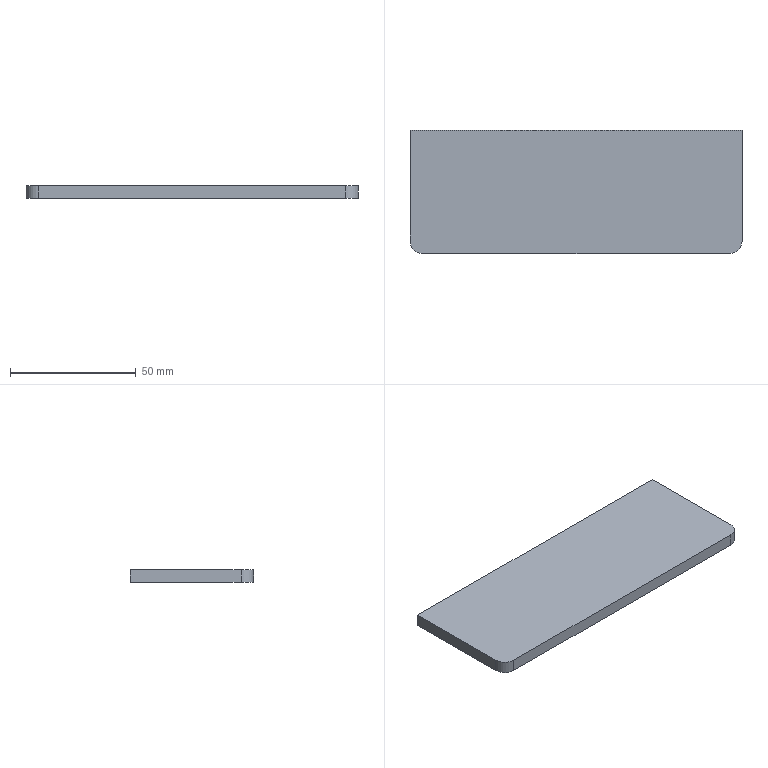Component | SolidWorks | LiftingVerticalBeamAssembly-1_LiftingVerticalBeamStiffener-2 | 1 solid | 8 faces | box 132 x 49 x 5 mm | volume 32286 mm3 | plane 6 | cylinder 2 | commonest cylinder face diameters 10 x2 | material Plain Carbon Steel
STEP:
#1=COLOUR_RGB('',0.7922,0.8196,0.9333);
#2=FILL_AREA_STYLE_COLOUR('',#1);
#3=FILL_AREA_STYLE('',(#2));
#4=SURFACE_STYLE_FILL_AREA(#3);
#5=SURFACE_SIDE_STYLE('',(#4));
#6=SURFACE_STYLE_USAGE(.BOTH.,#5);
#7=PRESENTATION_STYLE_ASSIGNMENT((#6));
#8=CARTESIAN_POINT('',(69.027,0.7303,53.05));
#9=VERTEX_POINT('',#8);
#10=CARTESIAN_POINT('',(69.027,-1.002,53.05));
#11=VERTEX_POINT('',#10);
#12=CARTESIAN_POINT('',(69.027,0.7303,53.05));
#13=DIRECTION('',(0.,-1.,0.));
#14=VECTOR('',#13,39.37);
#15=LINE('',#12,#14);
#16=EDGE_CURVE('',#9,#11,#15,.T.);
#17=ORIENTED_EDGE('',*,*,#16,.T.);
#18=CARTESIAN_POINT('',(69.027,-1.002,53.247));
#19=VERTEX_POINT('',#18);
#20=CARTESIAN_POINT('',(69.027,-1.002,53.05));
#21=DIRECTION('',(0.,0.,1.));
#22=VECTOR('',#21,39.37);
#23=LINE('',#20,#22);
#24=EDGE_CURVE('',#11,#19,#23,.T.);
#25=ORIENTED_EDGE('',*,*,#24,.T.);
#26=CARTESIAN_POINT('',(69.027,0.7303,53.247));
#27=VERTEX_POINT('',#26);
#28=CARTESIAN_POINT('',(69.027,0.7303,53.247));
#29=DIRECTION('',(0.,-1.,0.));
#30=VECTOR('',#29,39.37);
#31=LINE('',#28,#30);
#32=EDGE_CURVE('',#27,#19,#31,.T.);
#33=ORIENTED_EDGE('',*,*,#32,.F.);
#34=CARTESIAN_POINT('',(69.027,0.7303,53.05));
#35=DIRECTION('',(0.,0.,1.));
#36=VECTOR('',#35,39.37);
#37=LINE('',#34,#36);
#38=EDGE_CURVE('',#9,#27,#37,.T.);
#39=ORIENTED_EDGE('',*,*,#38,.F.);
#40=EDGE_LOOP('',(#17,#25,#33,#39));
#41=FACE_OUTER_BOUND('',#40,.T.);
#42=CARTESIAN_POINT('',(69.027,0.7303,53.05));
#43=DIRECTION('',(-1.,-0.,0.));
#44=DIRECTION('',(0.,-1.,0.));
#45=AXIS2_PLACEMENT_3D('',#42,#43,#44);
#46=PLANE('',#45);
#47=ADVANCED_FACE('',(#41),#46,.T.);
#48=CARTESIAN_POINT('',(74.224,0.7303,53.247));
#49=VERTEX_POINT('',#48);
#50=CARTESIAN_POINT('',(69.027,0.7303,53.247));
#51=DIRECTION('',(-1.,0.,0.));
#52=VECTOR('',#51,39.37);
#53=LINE('',#50,#52);
#54=EDGE_CURVE('',#49,#27,#53,.T.);
#55=ORIENTED_EDGE('',*,*,#54,.F.);
#56=CARTESIAN_POINT('',(74.224,0.7303,53.05));
#57=VERTEX_POINT('',#56);
#58=CARTESIAN_POINT('',(74.224,0.7303,53.05));
#59=DIRECTION('',(0.,0.,1.));
#60=VECTOR('',#59,39.37);
#61=LINE('',#58,#60);
#62=EDGE_CURVE('',#57,#49,#61,.T.);
#63=ORIENTED_EDGE('',*,*,#62,.F.);
#64=CARTESIAN_POINT('',(69.027,0.7303,53.05));
#65=DIRECTION('',(-1.,0.,0.));
#66=VECTOR('',#65,39.37);
#67=LINE('',#64,#66);
#68=EDGE_CURVE('',#57,#9,#67,.T.);
#69=ORIENTED_EDGE('',*,*,#68,.T.);
#70=ORIENTED_EDGE('',*,*,#38,.T.);
#71=EDGE_LOOP('',(#55,#63,#69,#70));
#72=FACE_OUTER_BOUND('',#71,.T.);
#73=CARTESIAN_POINT('',(69.027,0.7303,53.05));
#74=DIRECTION('',(0.,1.,0.));
#75=DIRECTION('',(0.,0.,1.));
#76=AXIS2_PLACEMENT_3D('',#73,#74,#75);
#77=PLANE('',#76);
#78=ADVANCED_FACE('',(#72),#77,.T.);
#79=CARTESIAN_POINT('',(74.224,-1.002,53.247));
#80=VERTEX_POINT('',#79);
#81=CARTESIAN_POINT('',(74.224,0.7303,53.247));
#82=DIRECTION('',(0.,1.,0.));
#83=VECTOR('',#82,39.37);
#84=LINE('',#81,#83);
#85=EDGE_CURVE('',#80,#49,#84,.T.);
#86=ORIENTED_EDGE('',*,*,#85,.F.);
#87=CARTESIAN_POINT('',(74.224,-1.002,53.05));
#88=VERTEX_POINT('',#87);
#89=CARTESIAN_POINT('',(74.224,-1.002,53.05));
#90=DIRECTION('',(0.,0.,-1.));
#91=VECTOR('',#90,39.37);
#92=LINE('',#89,#91);
#93=EDGE_CURVE('',#80,#88,#92,.T.);
#94=ORIENTED_EDGE('',*,*,#93,.T.);
#95=CARTESIAN_POINT('',(74.224,0.7303,53.05));
#96=DIRECTION('',(0.,1.,0.));
#97=VECTOR('',#96,39.37);
#98=LINE('',#95,#97);
#99=EDGE_CURVE('',#88,#57,#98,.T.);
#100=ORIENTED_EDGE('',*,*,#99,.T.);
#101=ORIENTED_EDGE('',*,*,#62,.T.);
#102=EDGE_LOOP('',(#86,#94,#100,#101));
#103=FACE_OUTER_BOUND('',#102,.T.);
#104=CARTESIAN_POINT('',(74.224,0.7303,53.05));
#105=DIRECTION('',(1.,0.,0.));
#106=DIRECTION('',(0.,0.,-1.));
#107=AXIS2_PLACEMENT_3D('',#104,#105,#106);
#108=PLANE('',#107);
#109=ADVANCED_FACE('',(#103),#108,.T.);
#110=CARTESIAN_POINT('',(69.224,-1.199,53.05));
#111=VERTEX_POINT('',#110);
#112=CARTESIAN_POINT('',(74.027,-1.199,53.05));
#113=VERTEX_POINT('',#112);
#114=CARTESIAN_POINT('',(69.027,-1.199,53.05));
#115=DIRECTION('',(1.,0.,0.));
#116=VECTOR('',#115,39.37);
#117=LINE('',#114,#116);
#118=EDGE_CURVE('',#111,#113,#117,.T.);
#119=ORIENTED_EDGE('',*,*,#118,.T.);
#120=CARTESIAN_POINT('',(74.027,-1.199,53.247));
#121=VERTEX_POINT('',#120);
#122=CARTESIAN_POINT('',(74.027,-1.199,53.05));
#123=DIRECTION('',(0.,0.,1.));
#124=VECTOR('',#123,39.37);
#125=LINE('',#122,#124);
#126=EDGE_CURVE('',#113,#121,#125,.T.);
#127=ORIENTED_EDGE('',*,*,#126,.T.);
#128=CARTESIAN_POINT('',(69.224,-1.199,53.247));
#129=VERTEX_POINT('',#128);
#130=CARTESIAN_POINT('',(69.027,-1.199,53.247));
#131=DIRECTION('',(1.,0.,0.));
#132=VECTOR('',#131,39.37);
#133=LINE('',#130,#132);
#134=EDGE_CURVE('',#129,#121,#133,.T.);
#135=ORIENTED_EDGE('',*,*,#134,.F.);
#136=CARTESIAN_POINT('',(69.224,-1.199,53.05));
#137=DIRECTION('',(0.,0.,-1.));
#138=VECTOR('',#137,39.37);
#139=LINE('',#136,#138);
#140=EDGE_CURVE('',#129,#111,#139,.T.);
#141=ORIENTED_EDGE('',*,*,#140,.T.);
#142=EDGE_LOOP('',(#119,#127,#135,#141));
#143=FACE_OUTER_BOUND('',#142,.T.);
#144=CARTESIAN_POINT('',(69.027,-1.199,53.05));
#145=DIRECTION('',(0.,-1.,0.));
#146=DIRECTION('',(0.,0.,-1.));
#147=AXIS2_PLACEMENT_3D('',#144,#145,#146);
#148=PLANE('',#147);
#149=ADVANCED_FACE('',(#143),#148,.T.);
#150=ORIENTED_EDGE('',*,*,#99,.F.);
#151=CARTESIAN_POINT('',(74.027,-1.002,53.05));
#152=DIRECTION('',(0.,0.,-1.));
#153=DIRECTION('',(1.,0.,0.));
#154=AXIS2_PLACEMENT_3D('',#151,#152,#153);
#155=CIRCLE('',#154,0.1969);
#156=EDGE_CURVE('',#88,#113,#155,.T.);
#157=ORIENTED_EDGE('',*,*,#156,.T.);
#158=ORIENTED_EDGE('',*,*,#118,.F.);
#159=CARTESIAN_POINT('',(69.224,-1.002,53.05));
#160=DIRECTION('',(0.,0.,-1.));
#161=DIRECTION('',(1.,0.,0.));
#162=AXIS2_PLACEMENT_3D('',#159,#160,#161);
#163=CIRCLE('',#162,0.1969);
#164=EDGE_CURVE('',#111,#11,#163,.T.);
#165=ORIENTED_EDGE('',*,*,#164,.T.);
#166=ORIENTED_EDGE('',*,*,#16,.F.);
#167=ORIENTED_EDGE('',*,*,#68,.F.);
#168=EDGE_LOOP('',(#150,#157,#158,#165,#166,#167));
#169=FACE_OUTER_BOUND('',#168,.T.);
#170=CARTESIAN_POINT('',(69.027,-1.199,53.05));
#171=DIRECTION('',(0.,0.,1.));
#172=DIRECTION('',(1.,0.,0.));
#173=AXIS2_PLACEMENT_3D('',#170,#171,#172);
#174=PLANE('',#173);
#175=ADVANCED_FACE('',(#169),#174,.F.);
#176=ORIENTED_EDGE('',*,*,#134,.T.);
#177=CARTESIAN_POINT('',(74.027,-1.002,53.247));
#178=DIRECTION('',(0.,0.,1.));
#179=DIRECTION('',(1.,0.,0.));
#180=AXIS2_PLACEMENT_3D('',#177,#178,#179);
#181=CIRCLE('',#180,0.1969);
#182=EDGE_CURVE('',#121,#80,#181,.T.);
#183=ORIENTED_EDGE('',*,*,#182,.T.);
#184=ORIENTED_EDGE('',*,*,#85,.T.);
#185=ORIENTED_EDGE('',*,*,#54,.T.);
#186=ORIENTED_EDGE('',*,*,#32,.T.);
#187=CARTESIAN_POINT('',(69.224,-1.002,53.247));
#188=DIRECTION('',(0.,0.,1.));
#189=DIRECTION('',(1.,0.,0.));
#190=AXIS2_PLACEMENT_3D('',#187,#188,#189);
#191=CIRCLE('',#190,0.1969);
#192=EDGE_CURVE('',#19,#129,#191,.T.);
#193=ORIENTED_EDGE('',*,*,#192,.T.);
#194=EDGE_LOOP('',(#176,#183,#184,#185,#186,#193));
#195=FACE_OUTER_BOUND('',#194,.T.);
#196=CARTESIAN_POINT('',(69.027,-1.199,53.247));
#197=DIRECTION('',(0.,0.,1.));
#198=DIRECTION('',(1.,0.,0.));
#199=AXIS2_PLACEMENT_3D('',#196,#197,#198);
#200=PLANE('',#199);
#201=ADVANCED_FACE('',(#195),#200,.T.);
#202=ORIENTED_EDGE('',*,*,#156,.F.);
#203=ORIENTED_EDGE('',*,*,#93,.F.);
#204=ORIENTED_EDGE('',*,*,#182,.F.);
#205=ORIENTED_EDGE('',*,*,#126,.F.);
#206=EDGE_LOOP('',(#202,#203,#204,#205));
#207=FACE_OUTER_BOUND('',#206,.T.);
#208=CARTESIAN_POINT('',(74.027,-1.002,53.05));
#209=DIRECTION('',(0.,0.,1.));
#210=DIRECTION('',(1.,0.,0.));
#211=AXIS2_PLACEMENT_3D('',#208,#209,#210);
#212=CYLINDRICAL_SURFACE('',#211,0.1969);
#213=ADVANCED_FACE('',(#207),#212,.T.);
#214=ORIENTED_EDGE('',*,*,#164,.F.);
#215=ORIENTED_EDGE('',*,*,#140,.F.);
#216=ORIENTED_EDGE('',*,*,#192,.F.);
#217=ORIENTED_EDGE('',*,*,#24,.F.);
#218=EDGE_LOOP('',(#214,#215,#216,#217));
#219=FACE_OUTER_BOUND('',#218,.T.);
#220=CARTESIAN_POINT('',(69.224,-1.002,53.05));
#221=DIRECTION('',(0.,0.,1.));
#222=DIRECTION('',(1.,0.,0.));
#223=AXIS2_PLACEMENT_3D('',#220,#221,#222);
#224=CYLINDRICAL_SURFACE('',#223,0.1969);
#225=ADVANCED_FACE('',(#219),#224,.T.);
#226=CLOSED_SHELL('',(#47,#78,#109,#149,#175,#201,#213,#225));
#227=MANIFOLD_SOLID_BREP('',#226);
#228=STYLED_ITEM('',(#7),#227);
#229=PRESENTATION_LAYER_ASSIGNMENT('','',(#228));
#230=(LENGTH_UNIT()NAMED_UNIT(*)SI_UNIT($,.METRE.));
#231=LENGTH_MEASURE_WITH_UNIT(LENGTH_MEASURE(0.0254),#230);
#232=DIMENSIONAL_EXPONENTS(1.,0.,0.,0.,0.,0.,0.);
#233=(CONVERSION_BASED_UNIT('',#231)LENGTH_UNIT()NAMED_UNIT(#232));
#234=UNCERTAINTY_MEASURE_WITH_UNIT(LENGTH_MEASURE(0.00001),#233,'','');
#235=(NAMED_UNIT(*)PLANE_ANGLE_UNIT()SI_UNIT($,.RADIAN.));
#236=(NAMED_UNIT(*)SI_UNIT($,.STERADIAN.)SOLID_ANGLE_UNIT());
#237=(GEOMETRIC_REPRESENTATION_CONTEXT(3)GLOBAL_UNCERTAINTY_ASSIGNED_CONTEXT((#234))GLOBAL_UNIT_ASSIGNED_CONTEXT((#233,#235,#236))REPRESENTATION_CONTEXT('',''));
#238=MECHANICAL_DESIGN_GEOMETRIC_PRESENTATION_REPRESENTATION('',(#228),#237);
#239=CARTESIAN_POINT('',(0.,0.,0.));
#240=DIRECTION('',(0.,0.,1.));
#241=DIRECTION('',(1.,0.,0.));
#242=AXIS2_PLACEMENT_3D('',#239,#240,#241);
#243=(LENGTH_UNIT()NAMED_UNIT(*)SI_UNIT($,.METRE.));
#244=LENGTH_MEASURE_WITH_UNIT(LENGTH_MEASURE(0.0254),#243);
#245=DIMENSIONAL_EXPONENTS(1.,0.,0.,0.,0.,0.,0.);
#246=(CONVERSION_BASED_UNIT('',#244)LENGTH_UNIT()NAMED_UNIT(#245));
#247=UNCERTAINTY_MEASURE_WITH_UNIT(LENGTH_MEASURE(0.00001),#246,'','');
#248=(NAMED_UNIT(*)PLANE_ANGLE_UNIT()SI_UNIT($,.RADIAN.));
#249=(NAMED_UNIT(*)SI_UNIT($,.STERADIAN.)SOLID_ANGLE_UNIT());
#250=(GEOMETRIC_REPRESENTATION_CONTEXT(3)GLOBAL_UNCERTAINTY_ASSIGNED_CONTEXT((#247))GLOBAL_UNIT_ASSIGNED_CONTEXT((#246,#248,#249))REPRESENTATION_CONTEXT('',''));
#251=ADVANCED_BREP_SHAPE_REPRESENTATION('',(#227,#242),#250);